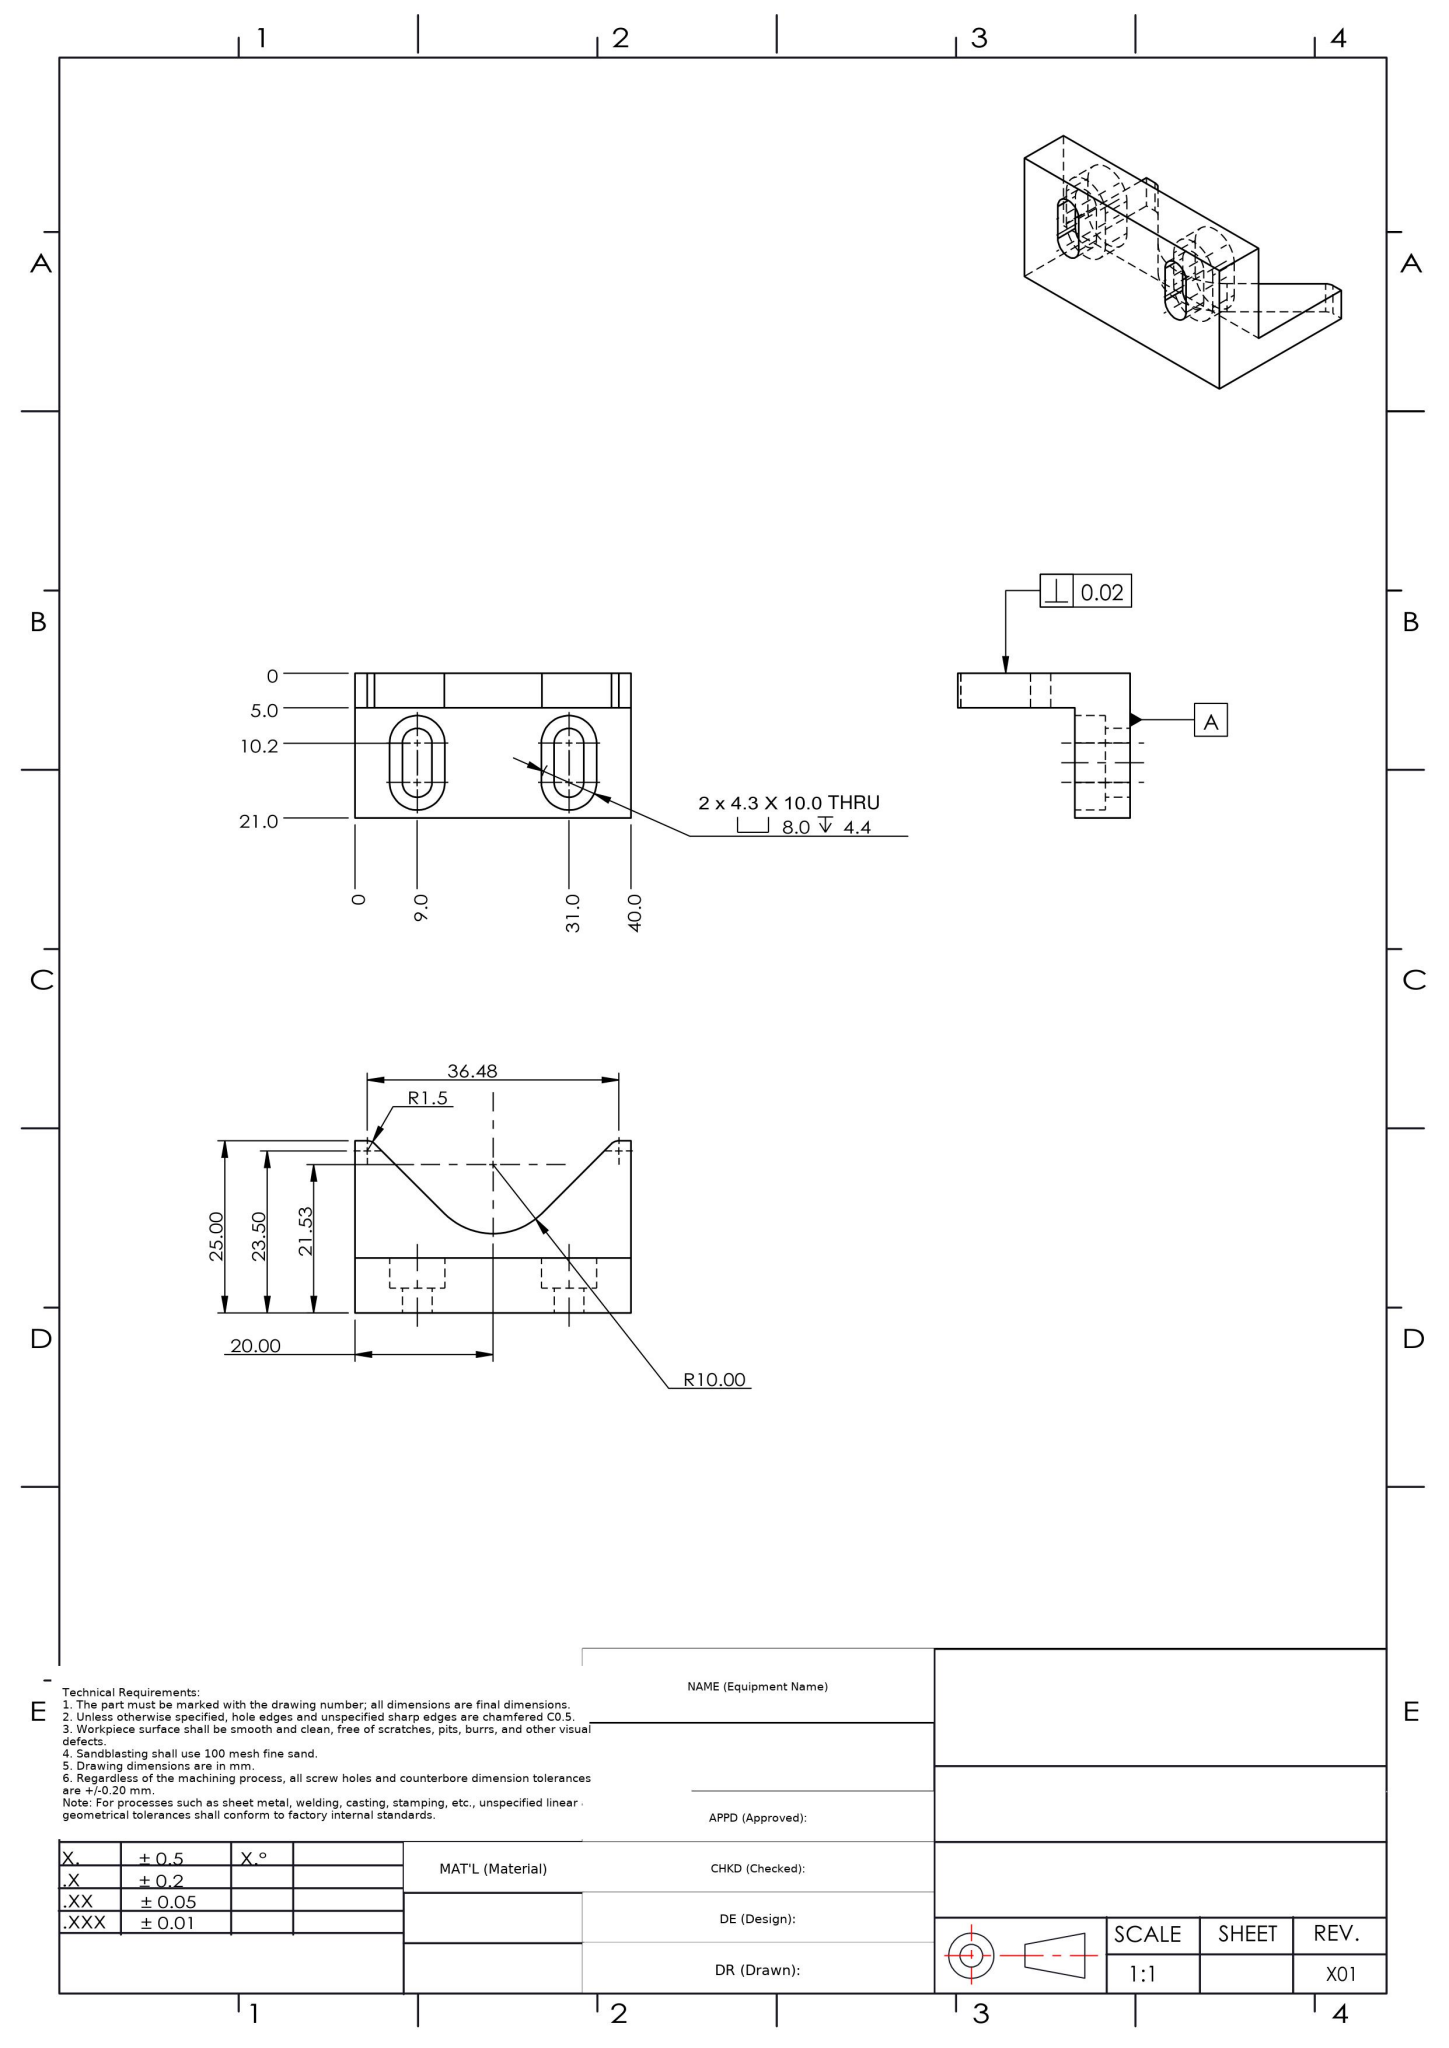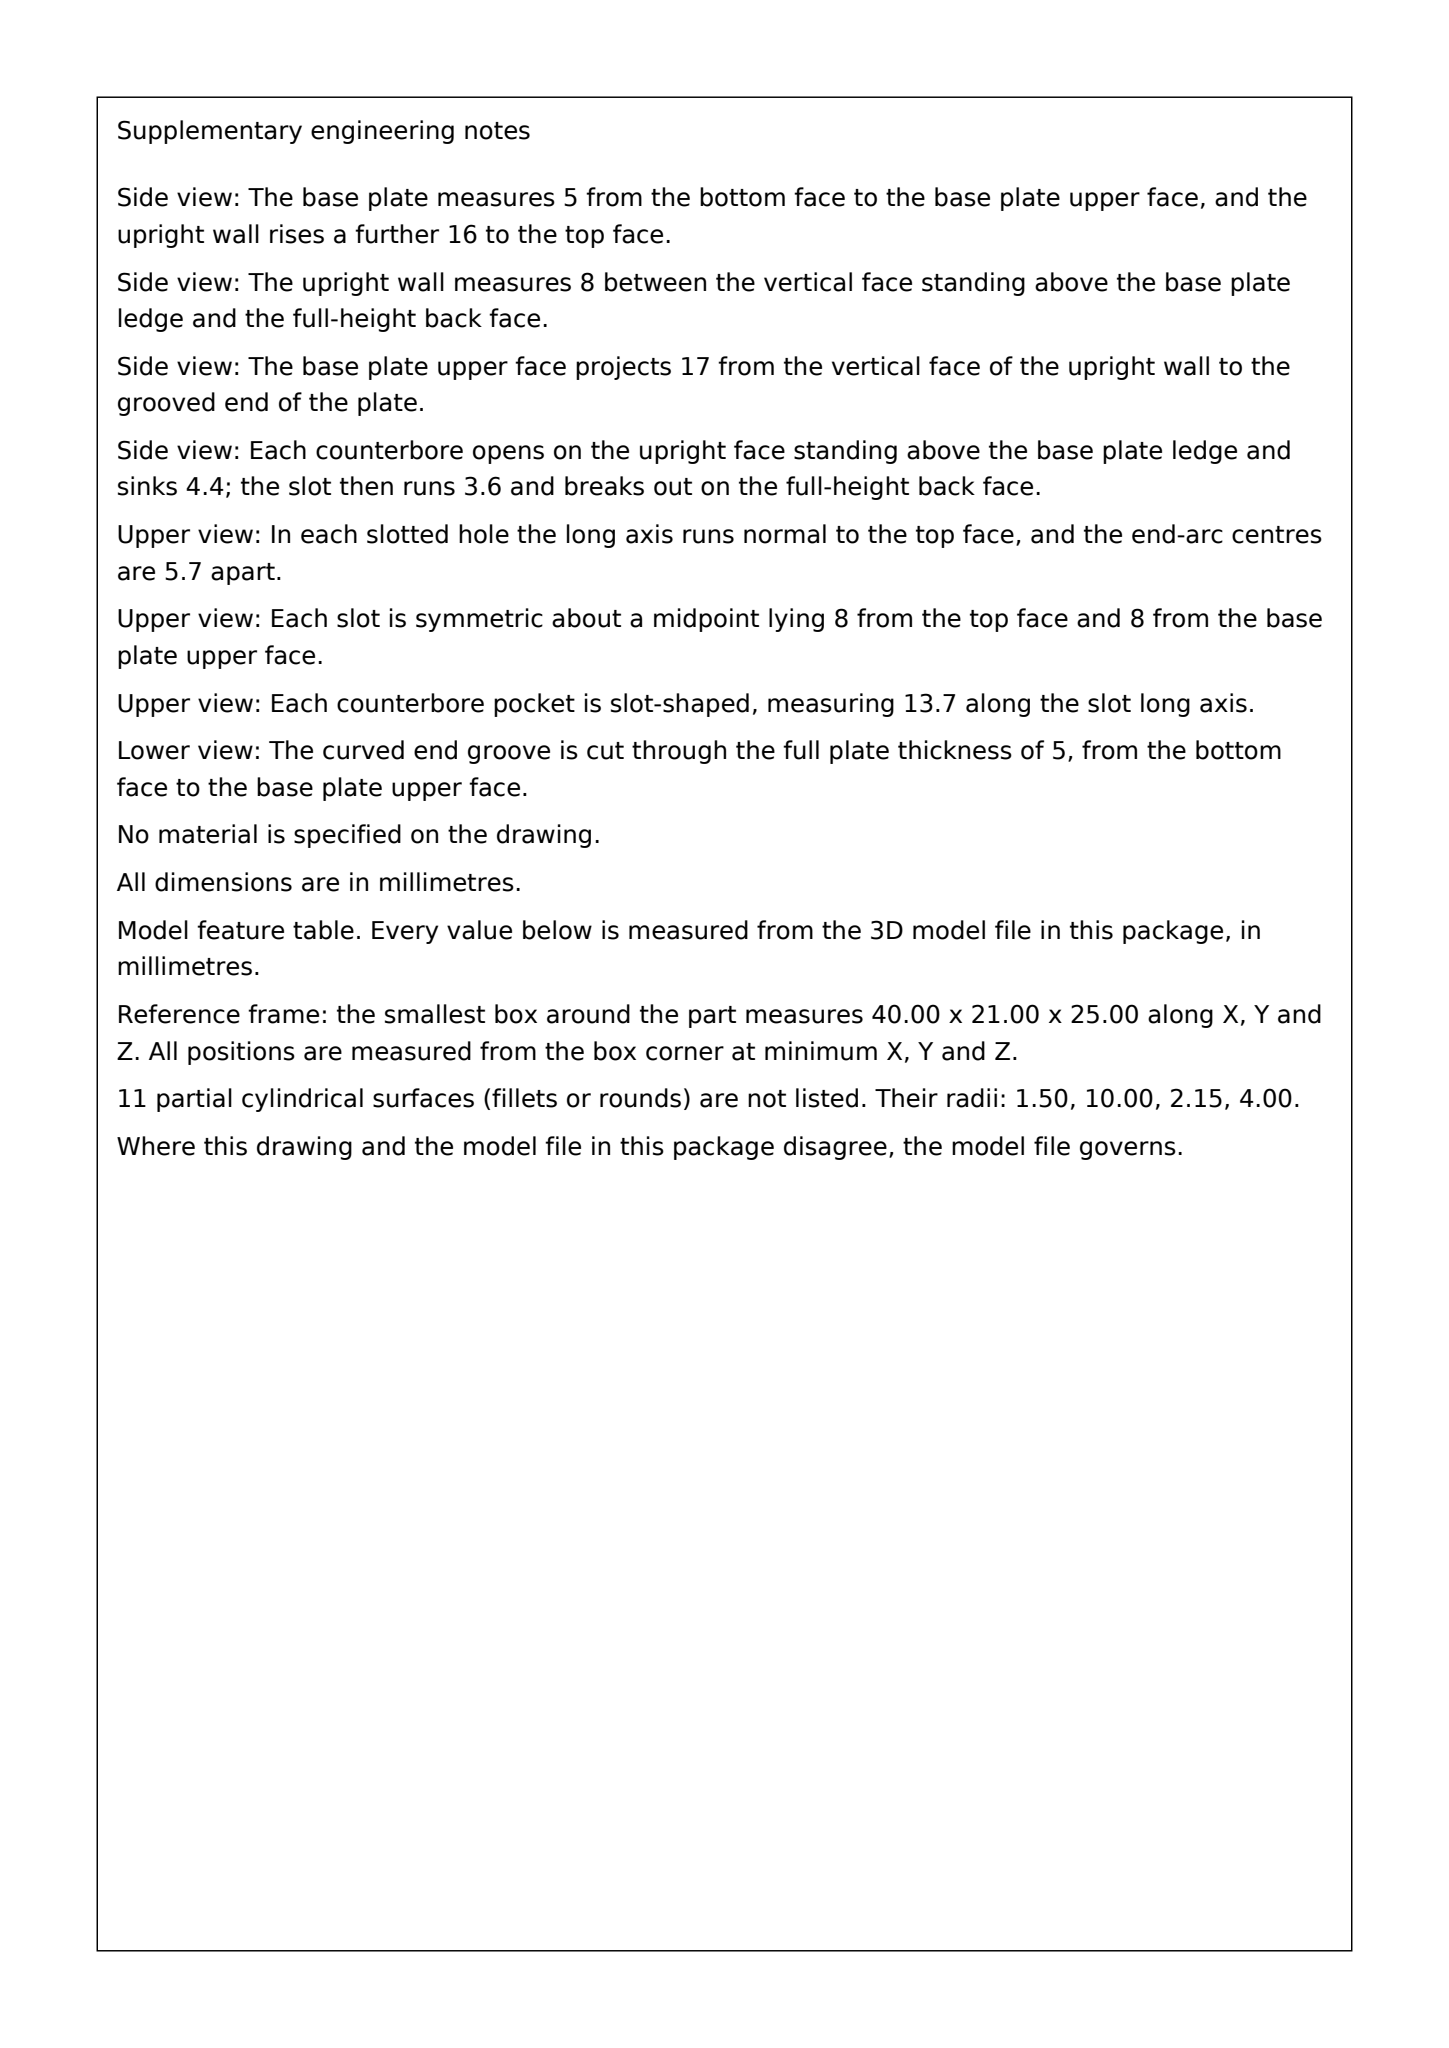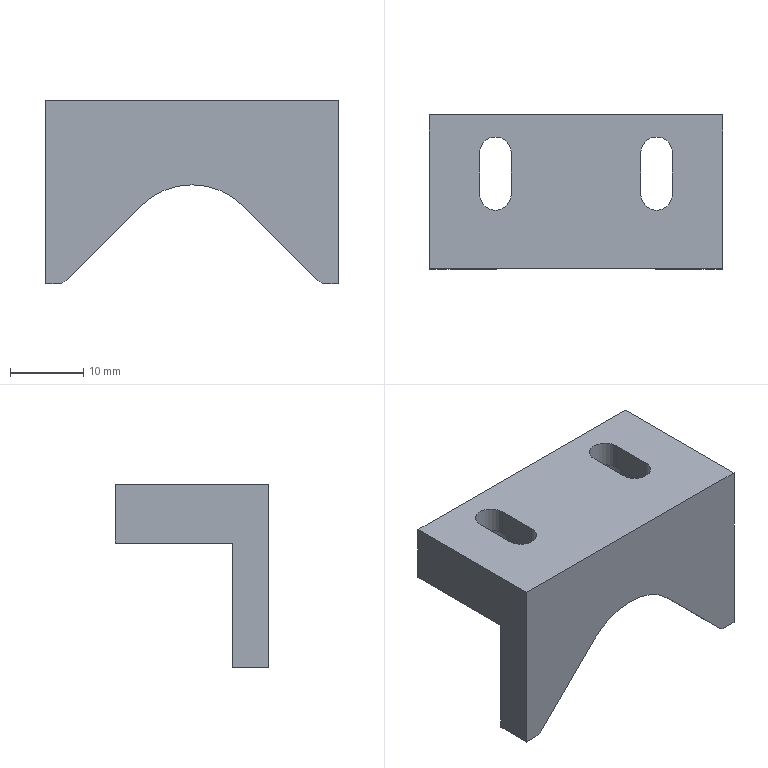Part | SolidWorks | mm | 1 solid | 32 faces | box 40 x 21 x 25 mm | volume 7550 mm3 | plane 21 | cylinder 11 | commonest cylinder face diameters 4.3 x4 8 x4 3 x2 20 x1